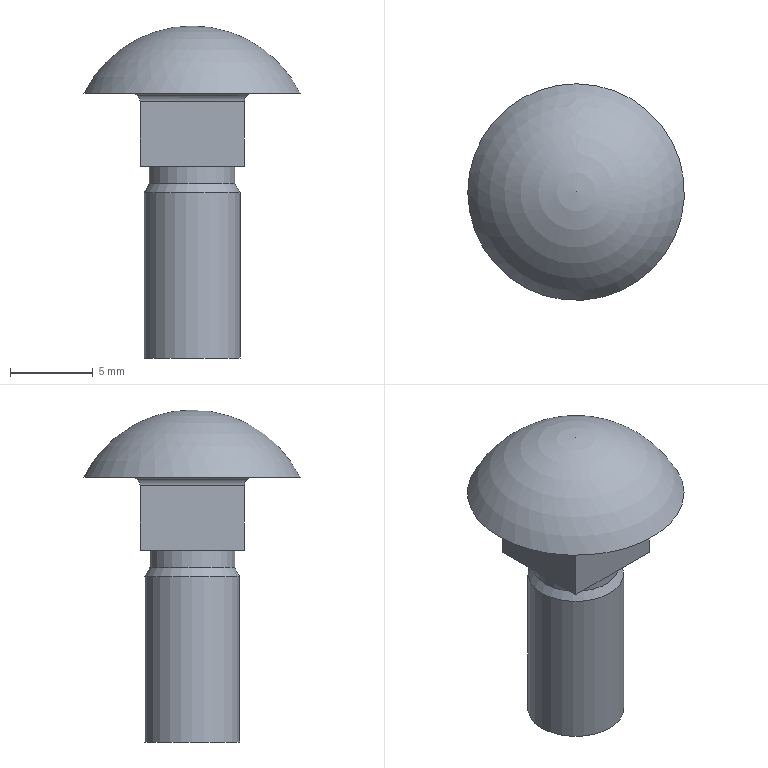Component | NX | GB12-88_M6X16 | 1 solid | 15 faces | volume 785 mm3 | plane 7 | cylinder 6 | cone 1 | sphere 1 | commonest cylinder face diameters 1 x4 5.183 x1 5.795 x1